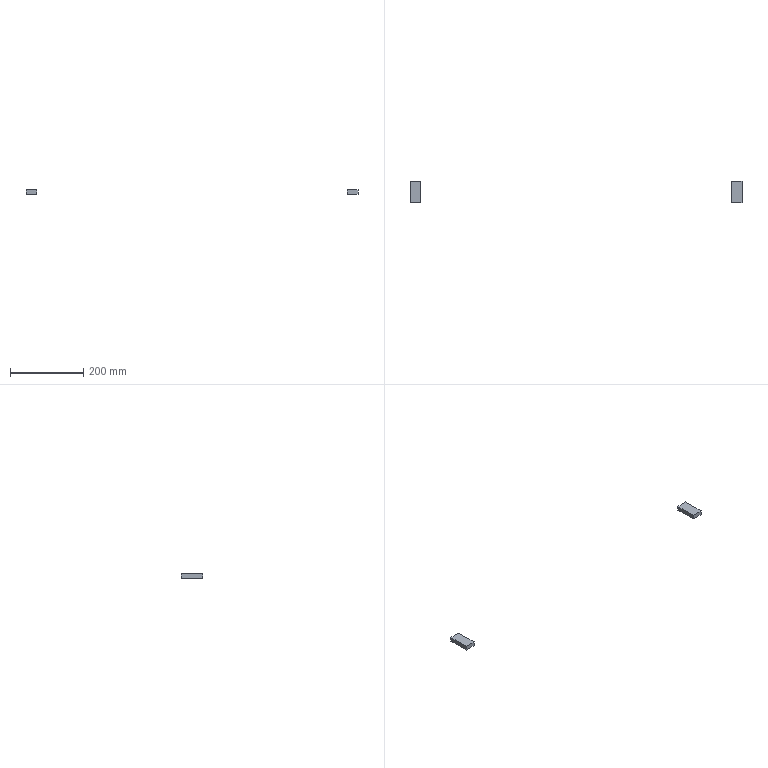Component | SolidWorks | Part2^SW-451-1 | 2 solids | 12 faces | box 909 x 60 x 12 mm | volume 43200 mm3 | plane 12
STEP:
#1=COLOUR_RGB('',0.7922,0.8196,0.9333);
#2=FILL_AREA_STYLE_COLOUR('',#1);
#3=FILL_AREA_STYLE('',(#2));
#4=SURFACE_STYLE_FILL_AREA(#3);
#5=SURFACE_SIDE_STYLE('',(#4));
#6=SURFACE_STYLE_USAGE(.BOTH.,#5);
#7=PRESENTATION_STYLE_ASSIGNMENT((#6));
#8=CARTESIAN_POINT('',(33.819,-2.362,4.123));
#9=VERTEX_POINT('',#8);
#10=CARTESIAN_POINT('',(35.,-2.362,4.123));
#11=VERTEX_POINT('',#10);
#12=CARTESIAN_POINT('',(-0.7874,-2.362,4.123));
#13=DIRECTION('',(1.,0.,0.));
#14=VECTOR('',#13,39.37);
#15=LINE('',#12,#14);
#16=EDGE_CURVE('',#9,#11,#15,.T.);
#17=ORIENTED_EDGE('',*,*,#16,.F.);
#18=CARTESIAN_POINT('',(33.819,-2.362,3.651));
#19=VERTEX_POINT('',#18);
#20=CARTESIAN_POINT('',(33.819,-2.362,4.123));
#21=DIRECTION('',(0.,0.,-1.));
#22=VECTOR('',#21,39.37);
#23=LINE('',#20,#22);
#24=EDGE_CURVE('',#9,#19,#23,.T.);
#25=ORIENTED_EDGE('',*,*,#24,.T.);
#26=CARTESIAN_POINT('',(35.,-2.362,3.651));
#27=VERTEX_POINT('',#26);
#28=CARTESIAN_POINT('',(-0.7874,-2.362,3.651));
#29=DIRECTION('',(1.,0.,0.));
#30=VECTOR('',#29,39.37);
#31=LINE('',#28,#30);
#32=EDGE_CURVE('',#19,#27,#31,.T.);
#33=ORIENTED_EDGE('',*,*,#32,.T.);
#34=CARTESIAN_POINT('',(35.,-2.362,4.123));
#35=DIRECTION('',(0.,0.,-1.));
#36=VECTOR('',#35,39.37);
#37=LINE('',#34,#36);
#38=EDGE_CURVE('',#11,#27,#37,.T.);
#39=ORIENTED_EDGE('',*,*,#38,.F.);
#40=EDGE_LOOP('',(#17,#25,#33,#39));
#41=FACE_OUTER_BOUND('',#40,.T.);
#42=CARTESIAN_POINT('',(-0.7874,-2.362,4.123));
#43=DIRECTION('',(0.,1.,0.));
#44=DIRECTION('',(0.,0.,1.));
#45=AXIS2_PLACEMENT_3D('',#42,#43,#44);
#46=PLANE('',#45);
#47=ADVANCED_FACE('',(#41),#46,.F.);
#48=CARTESIAN_POINT('',(35.,-0.,3.651));
#49=VERTEX_POINT('',#48);
#50=CARTESIAN_POINT('',(33.819,-0.,3.651));
#51=VERTEX_POINT('',#50);
#52=CARTESIAN_POINT('',(-0.7874,-0.,3.651));
#53=DIRECTION('',(-1.,0.,0.));
#54=VECTOR('',#53,39.37);
#55=LINE('',#52,#54);
#56=EDGE_CURVE('',#49,#51,#55,.T.);
#57=ORIENTED_EDGE('',*,*,#56,.T.);
#58=CARTESIAN_POINT('',(33.819,-0.,4.123));
#59=VERTEX_POINT('',#58);
#60=CARTESIAN_POINT('',(33.819,-0.,4.123));
#61=DIRECTION('',(0.,0.,-1.));
#62=VECTOR('',#61,39.37);
#63=LINE('',#60,#62);
#64=EDGE_CURVE('',#59,#51,#63,.T.);
#65=ORIENTED_EDGE('',*,*,#64,.F.);
#66=CARTESIAN_POINT('',(35.,-0.,4.123));
#67=VERTEX_POINT('',#66);
#68=CARTESIAN_POINT('',(-0.7874,-0.,4.123));
#69=DIRECTION('',(-1.,0.,0.));
#70=VECTOR('',#69,39.37);
#71=LINE('',#68,#70);
#72=EDGE_CURVE('',#67,#59,#71,.T.);
#73=ORIENTED_EDGE('',*,*,#72,.F.);
#74=CARTESIAN_POINT('',(35.,-0.,4.123));
#75=DIRECTION('',(0.,0.,-1.));
#76=VECTOR('',#75,39.37);
#77=LINE('',#74,#76);
#78=EDGE_CURVE('',#67,#49,#77,.T.);
#79=ORIENTED_EDGE('',*,*,#78,.T.);
#80=EDGE_LOOP('',(#57,#65,#73,#79));
#81=FACE_OUTER_BOUND('',#80,.T.);
#82=CARTESIAN_POINT('',(-0.7874,-0.,4.123));
#83=DIRECTION('',(0.,-1.,0.));
#84=DIRECTION('',(0.,0.,-1.));
#85=AXIS2_PLACEMENT_3D('',#82,#83,#84);
#86=PLANE('',#85);
#87=ADVANCED_FACE('',(#81),#86,.F.);
#88=ORIENTED_EDGE('',*,*,#72,.T.);
#89=CARTESIAN_POINT('',(33.819,-0.,4.123));
#90=DIRECTION('',(0.,-1.,0.));
#91=VECTOR('',#90,39.37);
#92=LINE('',#89,#91);
#93=EDGE_CURVE('',#59,#9,#92,.T.);
#94=ORIENTED_EDGE('',*,*,#93,.T.);
#95=ORIENTED_EDGE('',*,*,#16,.T.);
#96=CARTESIAN_POINT('',(35.,-2.362,4.123));
#97=DIRECTION('',(0.,1.,0.));
#98=VECTOR('',#97,39.37);
#99=LINE('',#96,#98);
#100=EDGE_CURVE('',#11,#67,#99,.T.);
#101=ORIENTED_EDGE('',*,*,#100,.T.);
#102=EDGE_LOOP('',(#88,#94,#95,#101));
#103=FACE_OUTER_BOUND('',#102,.T.);
#104=CARTESIAN_POINT('',(-0.7874,-2.362,4.123));
#105=DIRECTION('',(0.,0.,-1.));
#106=DIRECTION('',(-1.,0.,0.));
#107=AXIS2_PLACEMENT_3D('',#104,#105,#106);
#108=PLANE('',#107);
#109=ADVANCED_FACE('',(#103),#108,.F.);
#110=CARTESIAN_POINT('',(33.819,-0.,3.651));
#111=DIRECTION('',(0.,-1.,0.));
#112=VECTOR('',#111,39.37);
#113=LINE('',#110,#112);
#114=EDGE_CURVE('',#51,#19,#113,.T.);
#115=ORIENTED_EDGE('',*,*,#114,.F.);
#116=ORIENTED_EDGE('',*,*,#56,.F.);
#117=CARTESIAN_POINT('',(35.,-2.362,3.651));
#118=DIRECTION('',(0.,1.,0.));
#119=VECTOR('',#118,39.37);
#120=LINE('',#117,#119);
#121=EDGE_CURVE('',#27,#49,#120,.T.);
#122=ORIENTED_EDGE('',*,*,#121,.F.);
#123=ORIENTED_EDGE('',*,*,#32,.F.);
#124=EDGE_LOOP('',(#115,#116,#122,#123));
#125=FACE_OUTER_BOUND('',#124,.T.);
#126=CARTESIAN_POINT('',(-0.7874,-2.362,3.651));
#127=DIRECTION('',(0.,0.,-1.));
#128=DIRECTION('',(-1.,0.,0.));
#129=AXIS2_PLACEMENT_3D('',#126,#127,#128);
#130=PLANE('',#129);
#131=ADVANCED_FACE('',(#125),#130,.T.);
#132=ORIENTED_EDGE('',*,*,#121,.T.);
#133=ORIENTED_EDGE('',*,*,#78,.F.);
#134=ORIENTED_EDGE('',*,*,#100,.F.);
#135=ORIENTED_EDGE('',*,*,#38,.T.);
#136=EDGE_LOOP('',(#132,#133,#134,#135));
#137=FACE_OUTER_BOUND('',#136,.T.);
#138=CARTESIAN_POINT('',(35.,-2.362,4.123));
#139=DIRECTION('',(-1.,0.,0.));
#140=DIRECTION('',(0.,0.,1.));
#141=AXIS2_PLACEMENT_3D('',#138,#139,#140);
#142=PLANE('',#141);
#143=ADVANCED_FACE('',(#137),#142,.F.);
#144=ORIENTED_EDGE('',*,*,#114,.T.);
#145=ORIENTED_EDGE('',*,*,#24,.F.);
#146=ORIENTED_EDGE('',*,*,#93,.F.);
#147=ORIENTED_EDGE('',*,*,#64,.T.);
#148=EDGE_LOOP('',(#144,#145,#146,#147));
#149=FACE_OUTER_BOUND('',#148,.T.);
#150=CARTESIAN_POINT('',(33.819,-0.,4.123));
#151=DIRECTION('',(1.,0.,0.));
#152=DIRECTION('',(0.,0.,-1.));
#153=AXIS2_PLACEMENT_3D('',#150,#151,#152);
#154=PLANE('',#153);
#155=ADVANCED_FACE('',(#149),#154,.F.);
#156=CLOSED_SHELL('',(#47,#87,#109,#131,#143,#155));
#157=MANIFOLD_SOLID_BREP('',#156);
#158=STYLED_ITEM('',(#7),#157);
#159=PRESENTATION_LAYER_ASSIGNMENT('','',(#158));
#160=COLOUR_RGB('',0.7922,0.8196,0.9333);
#161=FILL_AREA_STYLE_COLOUR('',#160);
#162=FILL_AREA_STYLE('',(#161));
#163=SURFACE_STYLE_FILL_AREA(#162);
#164=SURFACE_SIDE_STYLE('',(#163));
#165=SURFACE_STYLE_USAGE(.BOTH.,#164);
#166=PRESENTATION_STYLE_ASSIGNMENT((#165));
#167=CARTESIAN_POINT('',(-0.7874,-0.,3.651));
#168=VERTEX_POINT('',#167);
#169=CARTESIAN_POINT('',(-0.7874,-2.362,3.651));
#170=VERTEX_POINT('',#169);
#171=CARTESIAN_POINT('',(-0.7874,-2.362,3.651));
#172=DIRECTION('',(0.,-1.,0.));
#173=VECTOR('',#172,39.37);
#174=LINE('',#171,#173);
#175=EDGE_CURVE('',#168,#170,#174,.T.);
#176=ORIENTED_EDGE('',*,*,#175,.T.);
#177=CARTESIAN_POINT('',(-0.7874,-2.362,4.123));
#178=VERTEX_POINT('',#177);
#179=CARTESIAN_POINT('',(-0.7874,-2.362,4.123));
#180=DIRECTION('',(0.,0.,-1.));
#181=VECTOR('',#180,39.37);
#182=LINE('',#179,#181);
#183=EDGE_CURVE('',#178,#170,#182,.T.);
#184=ORIENTED_EDGE('',*,*,#183,.F.);
#185=CARTESIAN_POINT('',(-0.7874,-0.,4.123));
#186=VERTEX_POINT('',#185);
#187=CARTESIAN_POINT('',(-0.7874,-2.362,4.123));
#188=DIRECTION('',(0.,-1.,0.));
#189=VECTOR('',#188,39.37);
#190=LINE('',#187,#189);
#191=EDGE_CURVE('',#186,#178,#190,.T.);
#192=ORIENTED_EDGE('',*,*,#191,.F.);
#193=CARTESIAN_POINT('',(-0.7874,-0.,4.123));
#194=DIRECTION('',(0.,0.,-1.));
#195=VECTOR('',#194,39.37);
#196=LINE('',#193,#195);
#197=EDGE_CURVE('',#186,#168,#196,.T.);
#198=ORIENTED_EDGE('',*,*,#197,.T.);
#199=EDGE_LOOP('',(#176,#184,#192,#198));
#200=FACE_OUTER_BOUND('',#199,.T.);
#201=CARTESIAN_POINT('',(-0.7874,-2.362,4.123));
#202=DIRECTION('',(1.,0.,0.));
#203=DIRECTION('',(0.,0.,-1.));
#204=AXIS2_PLACEMENT_3D('',#201,#202,#203);
#205=PLANE('',#204);
#206=ADVANCED_FACE('',(#200),#205,.F.);
#207=CARTESIAN_POINT('',(0.3937,-2.362,3.651));
#208=VERTEX_POINT('',#207);
#209=CARTESIAN_POINT('',(0.3937,-0.,3.651));
#210=VERTEX_POINT('',#209);
#211=CARTESIAN_POINT('',(0.3937,-0.,3.651));
#212=DIRECTION('',(0.,1.,0.));
#213=VECTOR('',#212,39.37);
#214=LINE('',#211,#213);
#215=EDGE_CURVE('',#208,#210,#214,.T.);
#216=ORIENTED_EDGE('',*,*,#215,.F.);
#217=CARTESIAN_POINT('',(-0.7874,-2.362,3.651));
#218=DIRECTION('',(1.,0.,0.));
#219=VECTOR('',#218,39.37);
#220=LINE('',#217,#219);
#221=EDGE_CURVE('',#170,#208,#220,.T.);
#222=ORIENTED_EDGE('',*,*,#221,.F.);
#223=ORIENTED_EDGE('',*,*,#175,.F.);
#224=CARTESIAN_POINT('',(-0.7874,-0.,3.651));
#225=DIRECTION('',(-1.,0.,0.));
#226=VECTOR('',#225,39.37);
#227=LINE('',#224,#226);
#228=EDGE_CURVE('',#210,#168,#227,.T.);
#229=ORIENTED_EDGE('',*,*,#228,.F.);
#230=EDGE_LOOP('',(#216,#222,#223,#229));
#231=FACE_OUTER_BOUND('',#230,.T.);
#232=CARTESIAN_POINT('',(-0.7874,-2.362,3.651));
#233=DIRECTION('',(0.,0.,-1.));
#234=DIRECTION('',(-1.,0.,0.));
#235=AXIS2_PLACEMENT_3D('',#232,#233,#234);
#236=PLANE('',#235);
#237=ADVANCED_FACE('',(#231),#236,.T.);
#238=CARTESIAN_POINT('',(0.3937,-2.362,4.123));
#239=VERTEX_POINT('',#238);
#240=CARTESIAN_POINT('',(-0.7874,-2.362,4.123));
#241=DIRECTION('',(1.,0.,0.));
#242=VECTOR('',#241,39.37);
#243=LINE('',#240,#242);
#244=EDGE_CURVE('',#178,#239,#243,.T.);
#245=ORIENTED_EDGE('',*,*,#244,.T.);
#246=CARTESIAN_POINT('',(0.3937,-0.,4.123));
#247=VERTEX_POINT('',#246);
#248=CARTESIAN_POINT('',(0.3937,-0.,4.123));
#249=DIRECTION('',(0.,1.,0.));
#250=VECTOR('',#249,39.37);
#251=LINE('',#248,#250);
#252=EDGE_CURVE('',#239,#247,#251,.T.);
#253=ORIENTED_EDGE('',*,*,#252,.T.);
#254=CARTESIAN_POINT('',(-0.7874,-0.,4.123));
#255=DIRECTION('',(-1.,0.,0.));
#256=VECTOR('',#255,39.37);
#257=LINE('',#254,#256);
#258=EDGE_CURVE('',#247,#186,#257,.T.);
#259=ORIENTED_EDGE('',*,*,#258,.T.);
#260=ORIENTED_EDGE('',*,*,#191,.T.);
#261=EDGE_LOOP('',(#245,#253,#259,#260));
#262=FACE_OUTER_BOUND('',#261,.T.);
#263=CARTESIAN_POINT('',(-0.7874,-2.362,4.123));
#264=DIRECTION('',(0.,0.,-1.));
#265=DIRECTION('',(-1.,0.,0.));
#266=AXIS2_PLACEMENT_3D('',#263,#264,#265);
#267=PLANE('',#266);
#268=ADVANCED_FACE('',(#262),#267,.F.);
#269=ORIENTED_EDGE('',*,*,#258,.F.);
#270=CARTESIAN_POINT('',(0.3937,-0.,4.123));
#271=DIRECTION('',(0.,0.,-1.));
#272=VECTOR('',#271,39.37);
#273=LINE('',#270,#272);
#274=EDGE_CURVE('',#247,#210,#273,.T.);
#275=ORIENTED_EDGE('',*,*,#274,.T.);
#276=ORIENTED_EDGE('',*,*,#228,.T.);
#277=ORIENTED_EDGE('',*,*,#197,.F.);
#278=EDGE_LOOP('',(#269,#275,#276,#277));
#279=FACE_OUTER_BOUND('',#278,.T.);
#280=CARTESIAN_POINT('',(-0.7874,-0.,4.123));
#281=DIRECTION('',(0.,-1.,0.));
#282=DIRECTION('',(0.,0.,-1.));
#283=AXIS2_PLACEMENT_3D('',#280,#281,#282);
#284=PLANE('',#283);
#285=ADVANCED_FACE('',(#279),#284,.F.);
#286=ORIENTED_EDGE('',*,*,#221,.T.);
#287=CARTESIAN_POINT('',(0.3937,-2.362,4.123));
#288=DIRECTION('',(0.,0.,-1.));
#289=VECTOR('',#288,39.37);
#290=LINE('',#287,#289);
#291=EDGE_CURVE('',#239,#208,#290,.T.);
#292=ORIENTED_EDGE('',*,*,#291,.F.);
#293=ORIENTED_EDGE('',*,*,#244,.F.);
#294=ORIENTED_EDGE('',*,*,#183,.T.);
#295=EDGE_LOOP('',(#286,#292,#293,#294));
#296=FACE_OUTER_BOUND('',#295,.T.);
#297=CARTESIAN_POINT('',(-0.7874,-2.362,4.123));
#298=DIRECTION('',(0.,1.,0.));
#299=DIRECTION('',(0.,0.,1.));
#300=AXIS2_PLACEMENT_3D('',#297,#298,#299);
#301=PLANE('',#300);
#302=ADVANCED_FACE('',(#296),#301,.F.);
#303=ORIENTED_EDGE('',*,*,#215,.T.);
#304=ORIENTED_EDGE('',*,*,#274,.F.);
#305=ORIENTED_EDGE('',*,*,#252,.F.);
#306=ORIENTED_EDGE('',*,*,#291,.T.);
#307=EDGE_LOOP('',(#303,#304,#305,#306));
#308=FACE_OUTER_BOUND('',#307,.T.);
#309=CARTESIAN_POINT('',(0.3937,-0.,4.123));
#310=DIRECTION('',(-1.,0.,0.));
#311=DIRECTION('',(0.,0.,1.));
#312=AXIS2_PLACEMENT_3D('',#309,#310,#311);
#313=PLANE('',#312);
#314=ADVANCED_FACE('',(#308),#313,.F.);
#315=CLOSED_SHELL('',(#206,#237,#268,#285,#302,#314));
#316=MANIFOLD_SOLID_BREP('',#315);
#317=STYLED_ITEM('',(#166),#316);
#318=(LENGTH_UNIT()NAMED_UNIT(*)SI_UNIT($,.METRE.));
#319=LENGTH_MEASURE_WITH_UNIT(LENGTH_MEASURE(0.0254),#318);
#320=DIMENSIONAL_EXPONENTS(1.,0.,0.,0.,0.,0.,0.);
#321=(CONVERSION_BASED_UNIT('',#319)LENGTH_UNIT()NAMED_UNIT(#320));
#322=UNCERTAINTY_MEASURE_WITH_UNIT(LENGTH_MEASURE(0.00001),#321,'','');
#323=(NAMED_UNIT(*)PLANE_ANGLE_UNIT()SI_UNIT($,.RADIAN.));
#324=(NAMED_UNIT(*)SI_UNIT($,.STERADIAN.)SOLID_ANGLE_UNIT());
#325=(GEOMETRIC_REPRESENTATION_CONTEXT(3)GLOBAL_UNCERTAINTY_ASSIGNED_CONTEXT((#322))GLOBAL_UNIT_ASSIGNED_CONTEXT((#321,#323,#324))REPRESENTATION_CONTEXT('',''));
#326=MECHANICAL_DESIGN_GEOMETRIC_PRESENTATION_REPRESENTATION('',(#317),#325);
#327=(LENGTH_UNIT()NAMED_UNIT(*)SI_UNIT($,.METRE.));
#328=LENGTH_MEASURE_WITH_UNIT(LENGTH_MEASURE(0.0254),#327);
#329=DIMENSIONAL_EXPONENTS(1.,0.,0.,0.,0.,0.,0.);
#330=(CONVERSION_BASED_UNIT('',#328)LENGTH_UNIT()NAMED_UNIT(#329));
#331=UNCERTAINTY_MEASURE_WITH_UNIT(LENGTH_MEASURE(0.00001),#330,'','');
#332=(NAMED_UNIT(*)PLANE_ANGLE_UNIT()SI_UNIT($,.RADIAN.));
#333=(NAMED_UNIT(*)SI_UNIT($,.STERADIAN.)SOLID_ANGLE_UNIT());
#334=(GEOMETRIC_REPRESENTATION_CONTEXT(3)GLOBAL_UNCERTAINTY_ASSIGNED_CONTEXT((#331))GLOBAL_UNIT_ASSIGNED_CONTEXT((#330,#332,#333))REPRESENTATION_CONTEXT('',''));
#335=MECHANICAL_DESIGN_GEOMETRIC_PRESENTATION_REPRESENTATION('',(#158),#334);
#336=CARTESIAN_POINT('',(0.,0.,0.));
#337=DIRECTION('',(0.,0.,1.));
#338=DIRECTION('',(1.,0.,0.));
#339=AXIS2_PLACEMENT_3D('',#336,#337,#338);
#340=(LENGTH_UNIT()NAMED_UNIT(*)SI_UNIT($,.METRE.));
#341=LENGTH_MEASURE_WITH_UNIT(LENGTH_MEASURE(0.0254),#340);
#342=DIMENSIONAL_EXPONENTS(1.,0.,0.,0.,0.,0.,0.);
#343=(CONVERSION_BASED_UNIT('',#341)LENGTH_UNIT()NAMED_UNIT(#342));
#344=UNCERTAINTY_MEASURE_WITH_UNIT(LENGTH_MEASURE(0.00001),#343,'','');
#345=(NAMED_UNIT(*)PLANE_ANGLE_UNIT()SI_UNIT($,.RADIAN.));
#346=(NAMED_UNIT(*)SI_UNIT($,.STERADIAN.)SOLID_ANGLE_UNIT());
#347=(GEOMETRIC_REPRESENTATION_CONTEXT(3)GLOBAL_UNCERTAINTY_ASSIGNED_CONTEXT((#344))GLOBAL_UNIT_ASSIGNED_CONTEXT((#343,#345,#346))REPRESENTATION_CONTEXT('',''));
#348=ADVANCED_BREP_SHAPE_REPRESENTATION('',(#157,#316,#339),#347);
#349=PRESENTATION_LAYER_ASSIGNMENT('','',(#317));